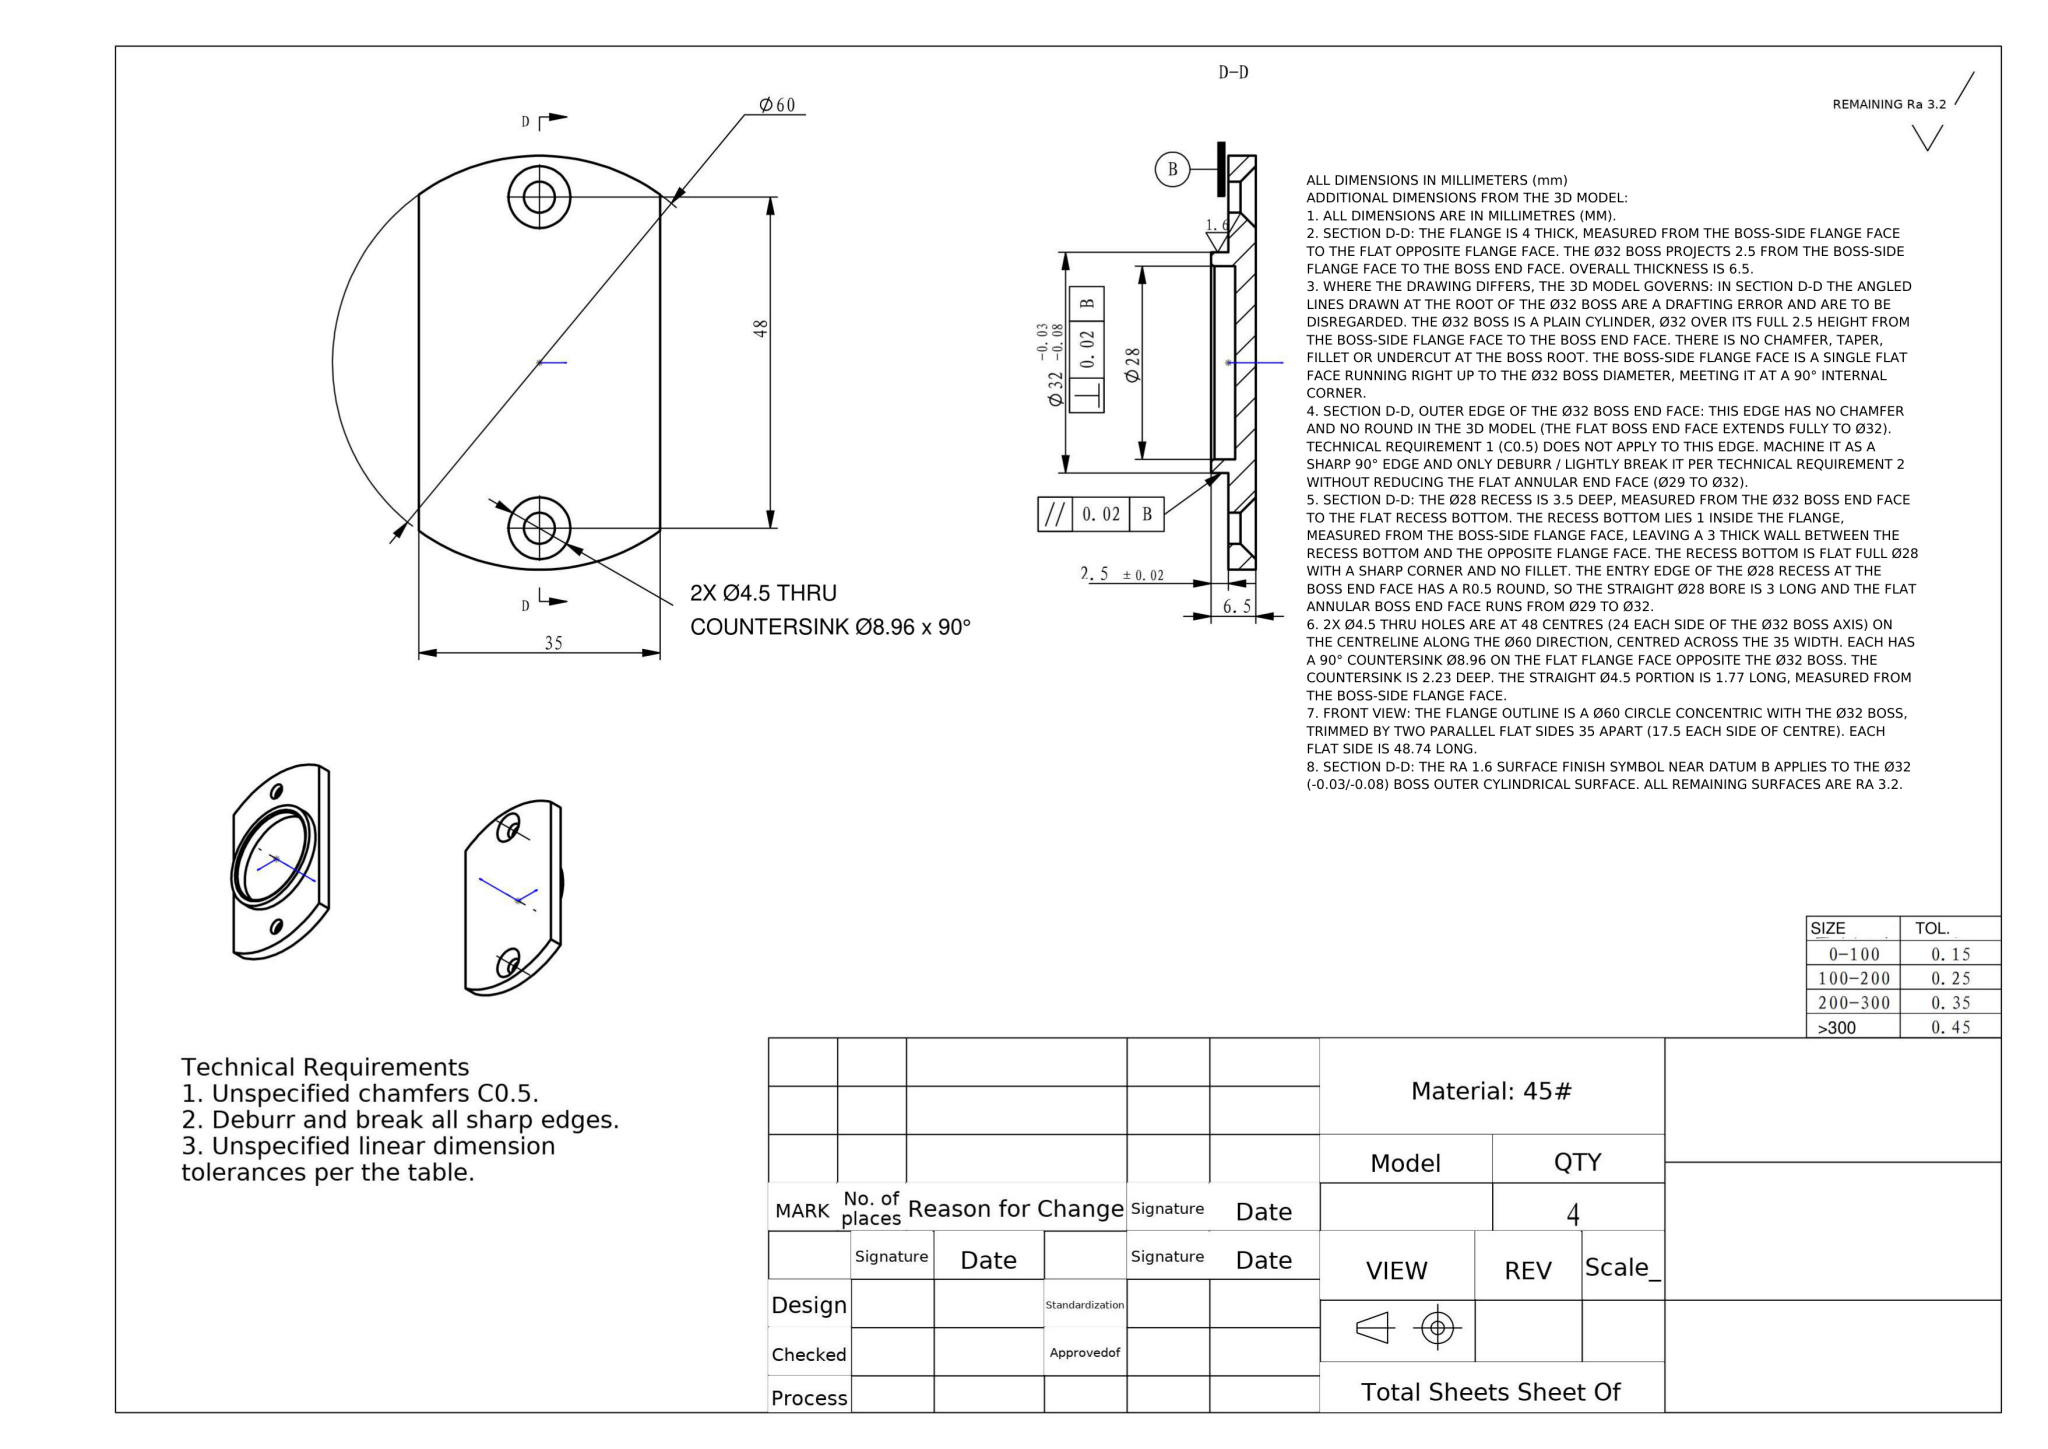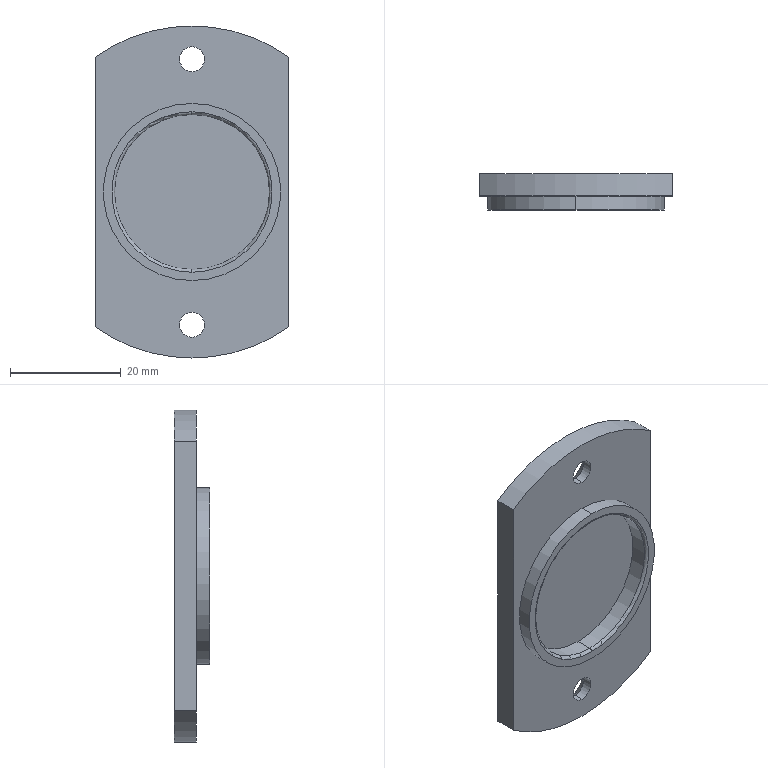Part | NX | mm | Arched Recessed Oval Mounting Plate | 1 solid | 23 faces | box 35 x 6.5 x 60 mm | volume 7526 mm3 | cylinder 11 | plane 6 | cone 4 | torus 2 | commonest cylinder face diameters 4.5 x4 60 x3 32 x2 28 x2